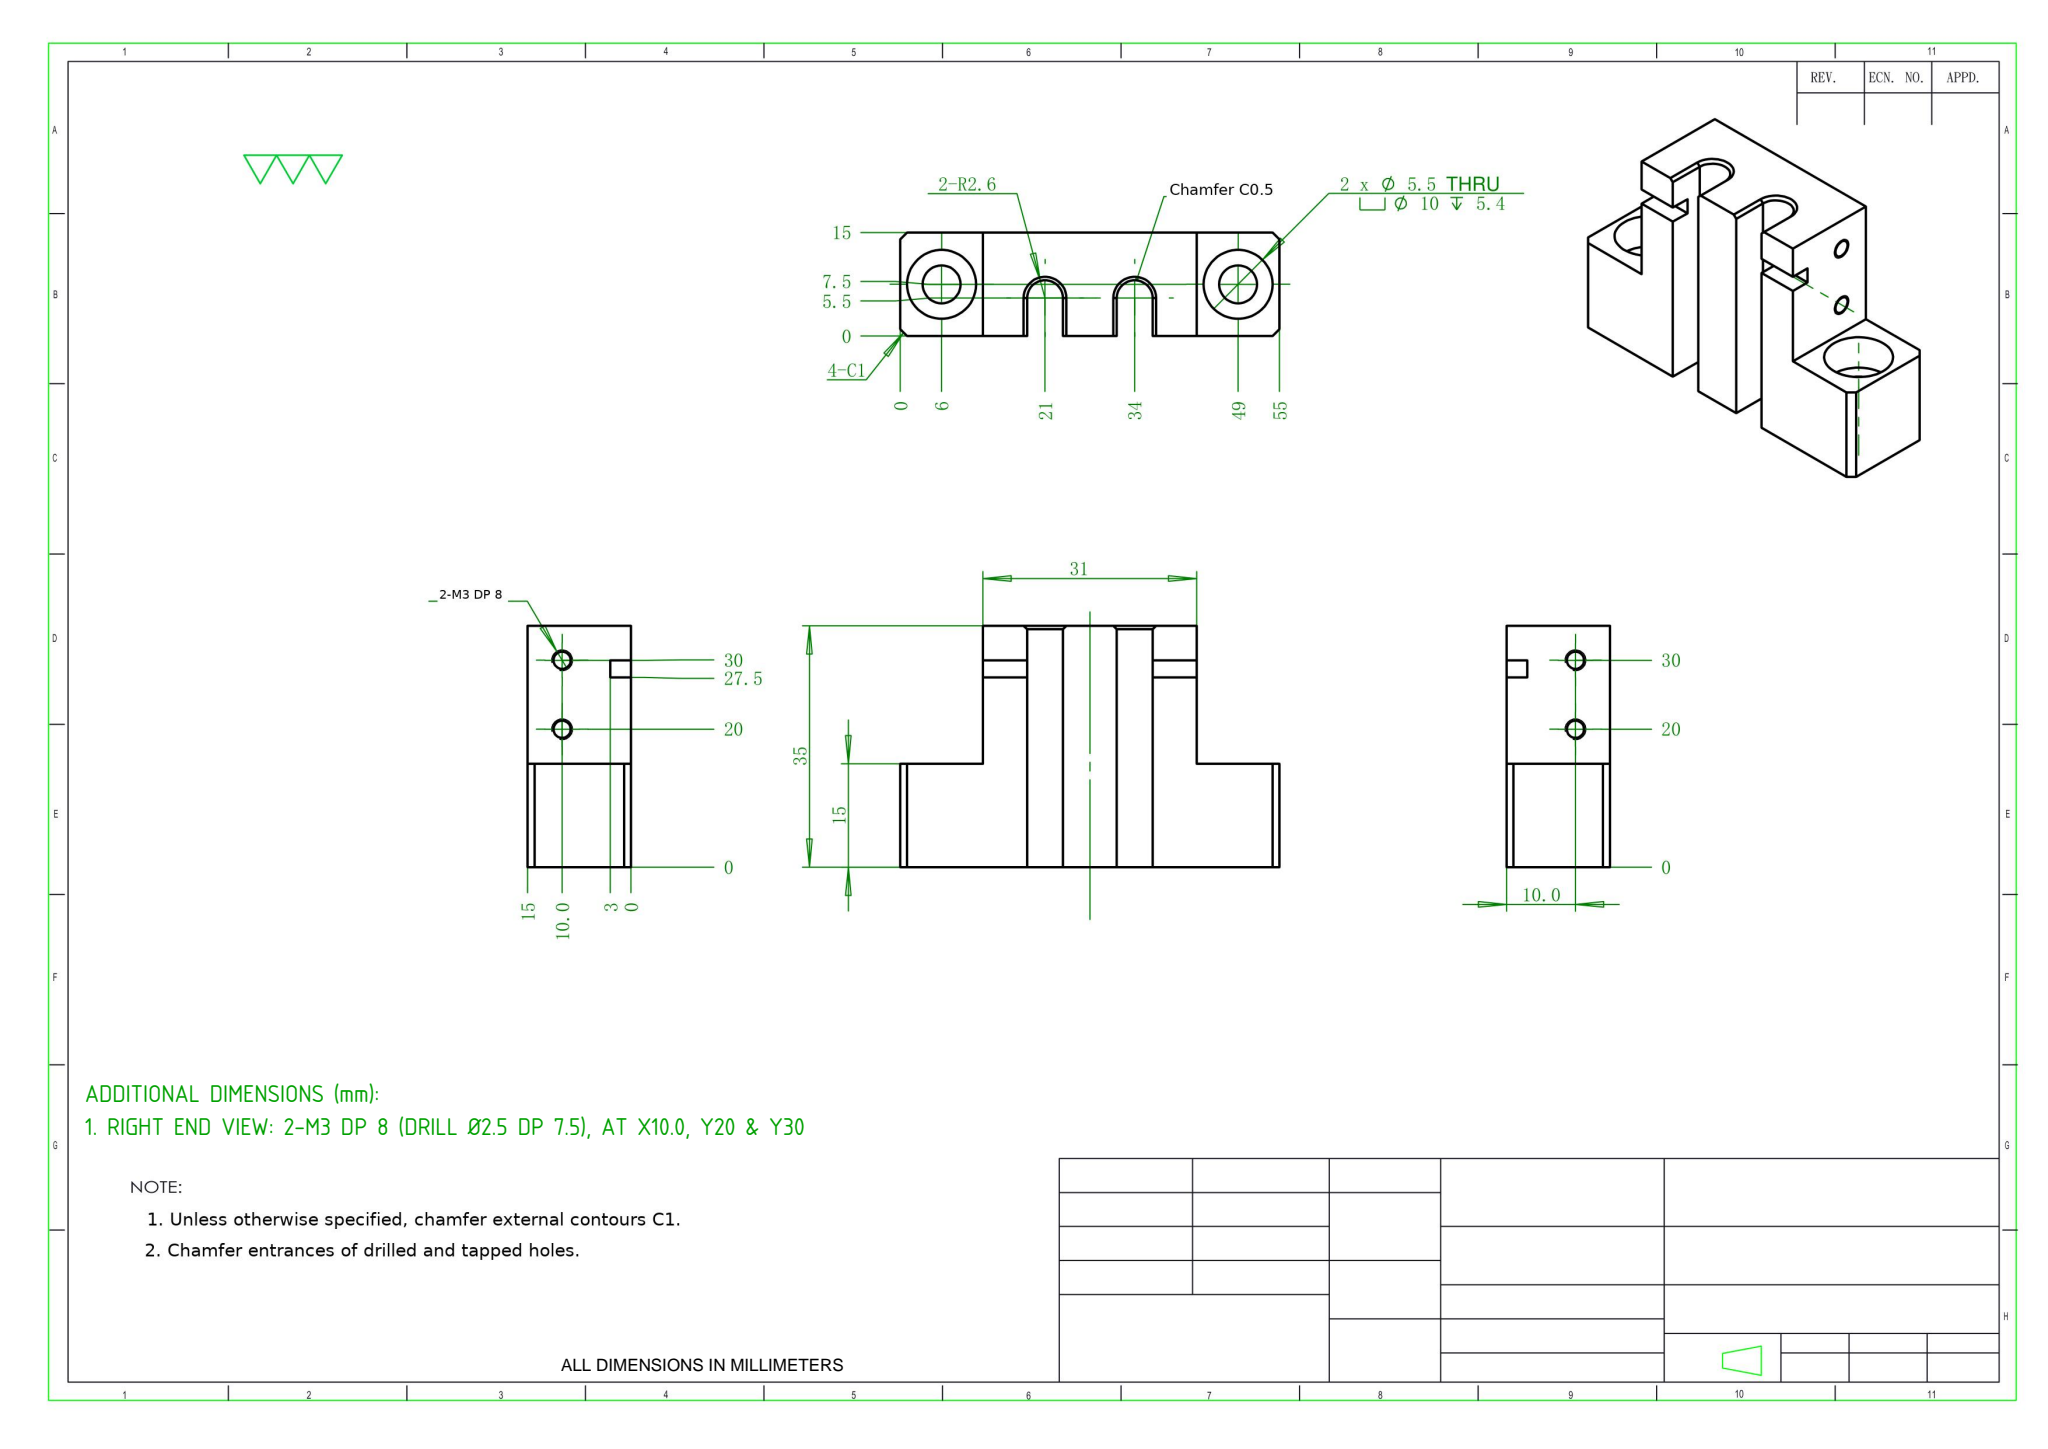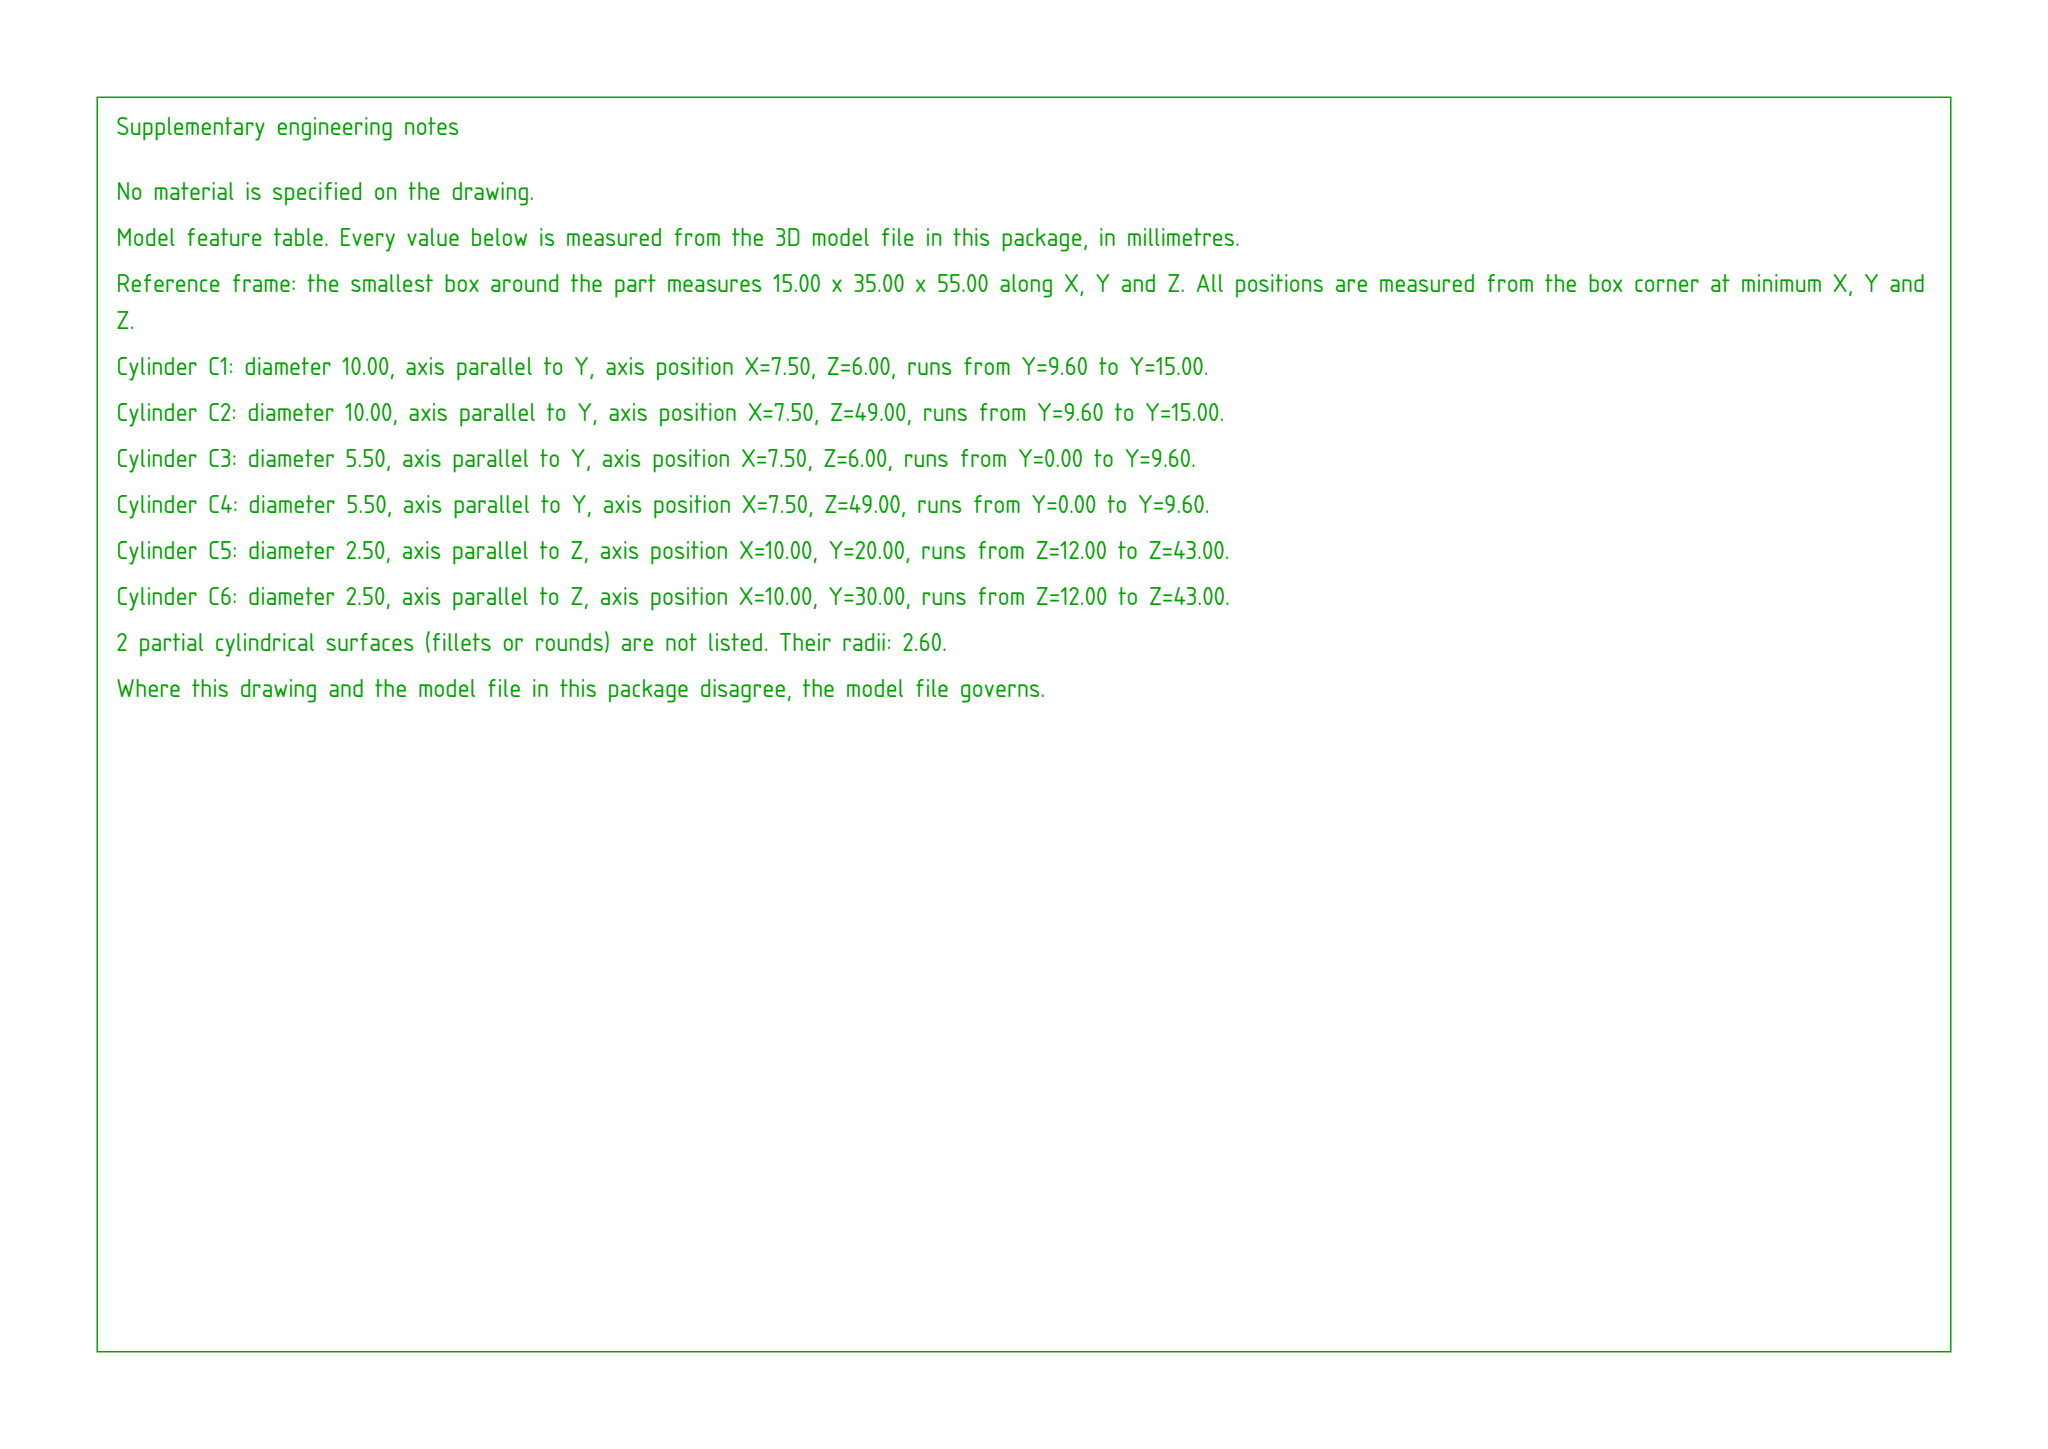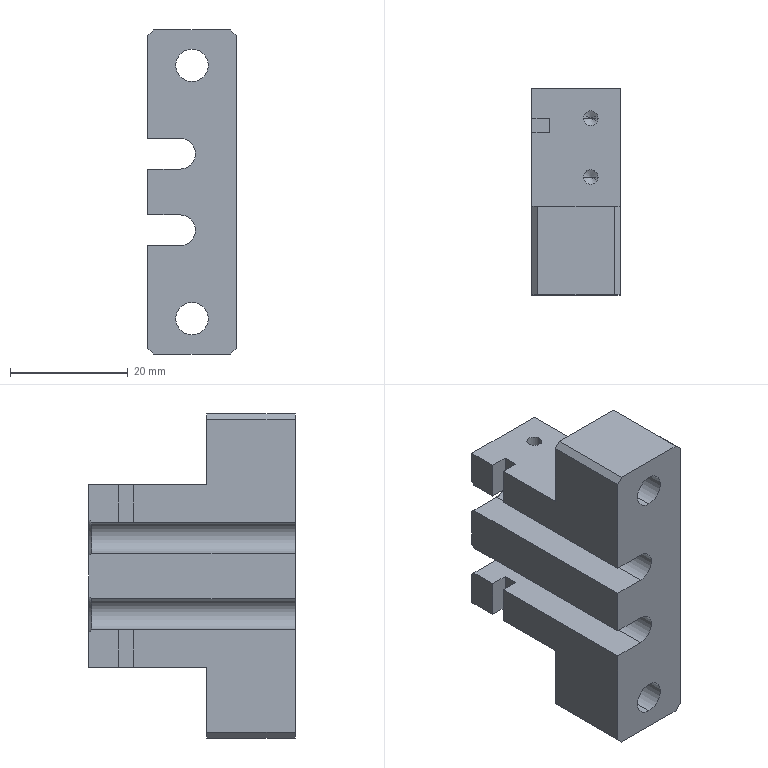Part | SolidWorks | mm | 1 solid | 62 faces | box 15 x 35 x 55 mm | volume 17342 mm3 | plane 34 | cylinder 18 | cone 10 | commonest cylinder face diameters 2.5 x8 10 x4 5.5 x4 5.2 x2
build123d program:
from build123d import *

# Parameters (mm, degrees)
SKETCH1_W                                       = 15
SKETCH1_H                                       = 55
BOSS_EXTRUDE1_DEPTH                             = 35
CUT_EXTRUDE1_DEPTH                              = 46.139
SKETCH8_W                                       = 15
SKETCH8_H                                       = 12
CUT_EXTRUDE2_DEPTH                              = 20
SKETCH9_W                                       = 6.4
SKETCH9_H                                       = 2.5
CUT_EXTRUDE3_DEPTH                              = 3
M3_TAPPED_HOLE1_AT_2_COUNT                      = 2
M3_TAPPED_HOLE1_AT_2_PITCH                      = 10
CHAMFER1_SIZE                                   = 0.5
M5_HEX_SOCKET_HEAD_CAP_SCREW_CBORE1_D           = 5.5
M5_HEX_SOCKET_HEAD_CAP_SCREW_CBORE1_CBORE_D     = 10
M5_HEX_SOCKET_HEAD_CAP_SCREW_CBORE1_CBORE_DEPTH = 5.4
CHAMFER2_SIZE                                   = 1


with BuildPart() as part:
    # Sketch1 → Boss-Extrude1 (new body)
    with BuildSketch(Plane(origin=(0, 0, 0), x_dir=(1, 0, 0), z_dir=(0, 1, 0))):
        Rectangle(SKETCH1_W, SKETCH1_H)
    extrude(amount=BOSS_EXTRUDE1_DEPTH)

    # Sketch7 → Cut-Extrude1 (cut, through all)
    with BuildSketch(Plane(origin=(0, 35, 0), x_dir=(1, 0, 0), z_dir=(0, 1, 0))):
        with BuildLine():
            Line((-7.5, 9.1), (-2, 9.1))
            ThreePointArc((-2, 9.1), (0.6, 6.5), (-2, 3.9))
            Line((-2, 3.9), (-7.5, 3.9))
            ThreePointArc((-7.5, 3.9), (-10.1, 6.5), (-7.5, 9.1))
        make_face()
        with BuildLine():
            Line((-7.5, -9.1), (-2, -9.1))
            ThreePointArc((-2, -9.1), (0.6, -6.5), (-2, -3.9))
            Line((-2, -3.9), (-7.5, -3.9))
            ThreePointArc((-7.5, -3.9), (-10.1, -6.5), (-7.5, -9.1))
        make_face()
    extrude(amount=-CUT_EXTRUDE1_DEPTH, mode=Mode.SUBTRACT)

    # Sketch8 → Cut-Extrude2 (cut)
    with BuildSketch(Plane(origin=(0, 35, 0), x_dir=(1, 0, 0), z_dir=(0, 1, 0))):
        with Locations((0, 21.5)):
            Rectangle(SKETCH8_W, SKETCH8_H)
        with Locations((0, -21.5)):
            Rectangle(SKETCH8_W, SKETCH8_H)
    extrude(amount=-CUT_EXTRUDE2_DEPTH, mode=Mode.SUBTRACT)

    # Sketch9 → Cut-Extrude3 (cut)
    with BuildSketch(Plane.ZY.offset(7.5)):
        with Locations((-12.3, 28.75)):
            Rectangle(SKETCH9_W, SKETCH9_H)
        with Locations((12.3, 28.75)):
            Rectangle(SKETCH9_W, SKETCH9_H)
    extrude(amount=-CUT_EXTRUDE3_DEPTH, mode=Mode.SUBTRACT)

    # Sketch10 → M3 Tapped Hole1 (revolve, cut)
    with BuildSketch(Plane(origin=(2.5, 30, -15.5), x_dir=(0, 1, 0), z_dir=(1, 0, 0))):
        Polygon((0, 0), (0, 8.251), (1.25, 7.5), (1.25, 0), align=None)
    m3_tapped_hole1 = revolve(axis=Axis((2.5, 30, -21.85), (0, 0, 1)), mode=Mode.SUBTRACT)

    # M3 Tapped Hole1 at 2: M3 Tapped Hole1 ×2
    with Locations(*[(0, -i * M3_TAPPED_HOLE1_AT_2_PITCH, 0) for i in range(1, M3_TAPPED_HOLE1_AT_2_COUNT)]):
        add(m3_tapped_hole1, mode=Mode.SUBTRACT)

    # Chamfer1
    chamfer1_edges = [part.edges().sort_by_distance(p)[0] for p in [
        (-4.75, 35, -9.1),
        (-4.75, 35, -3.9),
        (0.6, 35, -6.5),
        (-4.75, 35, 9.1),
        (0.6, 35, 6.5),
        (-4.75, 35, 3.9),
    ]]
    chamfer(chamfer1_edges, length=CHAMFER1_SIZE)

    # M5 Hex Socket Head Cap Screw CBORE1 (through all)
    with Locations(Plane(origin=(0, 15, 0), x_dir=(1, 0, 0), z_dir=(0, 1, 0))):
        with Locations((0, 21.5), (0, -21.5)):
            CounterBoreHole(M5_HEX_SOCKET_HEAD_CAP_SCREW_CBORE1_D / 2, M5_HEX_SOCKET_HEAD_CAP_SCREW_CBORE1_CBORE_D / 2, M5_HEX_SOCKET_HEAD_CAP_SCREW_CBORE1_CBORE_DEPTH)

    # Chamfer2
    chamfer2_edges = [part.edges().sort_by_distance(p)[0] for p in [
        (-7.5, 7.5, -27.5),
        (7.5, 7.5, -27.5),
        (7.5, 7.5, 27.5),
        (-7.5, 7.5, 27.5),
    ]]
    chamfer(chamfer2_edges, length=CHAMFER2_SIZE)

    # Mirror1: M3 Tapped Hole1 across plane
    add(m3_tapped_hole1.mirror(Plane.XY), mode=Mode.SUBTRACT)

    # Mirror1 copy 1 sketch → Mirror1 copy 1 (revolve, cut)
    with BuildSketch(Plane(origin=(2.5, 20, 15.5), x_dir=(0, 1, 0), z_dir=(1, 0, 0))):
        Polygon((0, 0), (0, -8.251), (1.25, -7.5), (1.25, 0), align=None)
    revolve(axis=Axis((2.5, 20, 21.85), (0, 0, 1)), mode=Mode.SUBTRACT)


solid = part.part